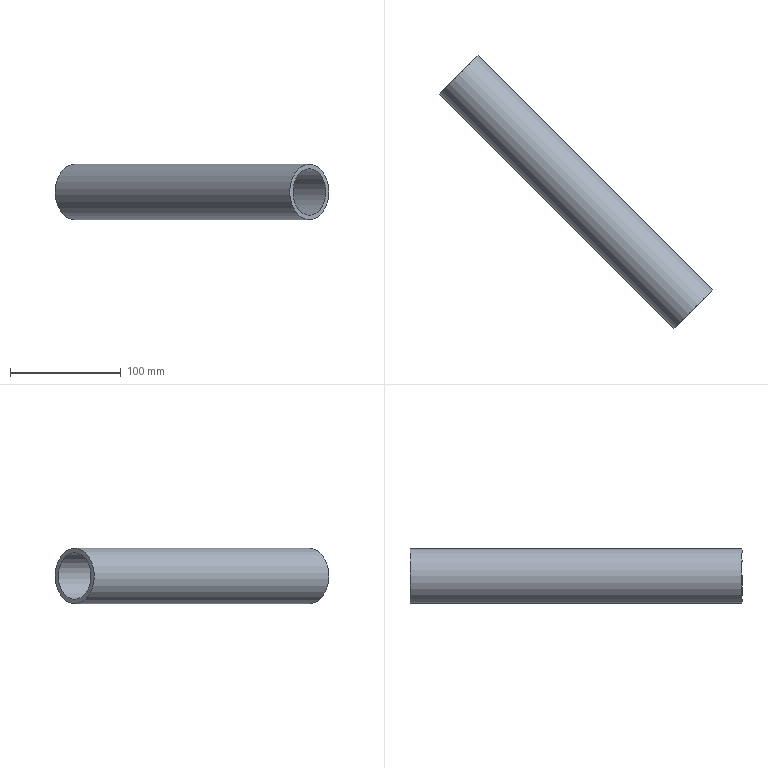Component | NX | SLID_FRAME_CONN_COL2 | 1 solid | 4 faces | box 247.49 x 247.49 x 50 mm | volume 173416 mm3 | cylinder 2 | plane 2 | commonest cylinder face diameters 50 x1 42 x1
STEP:
#1=CARTESIAN_POINT('',(0.,0.,0.));
#2=DIRECTION('',(0.,0.,1.));
#3=DIRECTION('',(1.,0.,0.));
#4=AXIS2_PLACEMENT_3D('',#1,#2,#3);
#5=CARTESIAN_POINT('',(-900.214,1525.378,235.));
#6=VERTEX_POINT('',#5);
#7=CARTESIAN_POINT('',(-900.214,1525.378,260.));
#8=DIRECTION('',(0.7071,-0.7071,0.));
#9=DIRECTION('',(0.,0.,-1.));
#10=AXIS2_PLACEMENT_3D('',#7,#8,#9);
#11=CIRCLE('',#10,25.);
#12=CARTESIAN_POINT('',(-900.214,1525.378,260.));
#13=DIRECTION('',(0.7071,-0.7071,0.));
#14=DIRECTION('',(0.,0.,1.));
#15=AXIS2_PLACEMENT_3D('',#12,#13,#14);
#16=CYLINDRICAL_SURFACE('',#15,25.);
#17=CARTESIAN_POINT('',(3.142,0.));
#18=DIRECTION('',(1.,0.));
#19=VECTOR('',#18,1.);
#20=LINE('',#17,#19);
#21=(GEOMETRIC_REPRESENTATION_CONTEXT(2)PARAMETRIC_REPRESENTATION_CONTEXT()REPRESENTATION_CONTEXT('',''));
#22=DEFINITIONAL_REPRESENTATION('',(#20),#21);
#23=PCURVE('',#16,#22);
#24=CARTESIAN_POINT('',(-900.214,1525.378,260.));
#25=DIRECTION('',(0.7071,-0.7071,0.));
#26=DIRECTION('',(0.,0.,1.));
#27=AXIS2_PLACEMENT_3D('',#24,#25,#26);
#28=PLANE('',#27);
#29=CARTESIAN_POINT('',(0.,0.));
#30=DIRECTION('',(-1.,0.));
#31=AXIS2_PLACEMENT_2D('',#29,#30);
#32=CIRCLE('',#31,25.);
#33=(GEOMETRIC_REPRESENTATION_CONTEXT(2)PARAMETRIC_REPRESENTATION_CONTEXT()REPRESENTATION_CONTEXT('',''));
#34=DEFINITIONAL_REPRESENTATION('',(#32),#33);
#35=PCURVE('',#28,#34);
#36=SURFACE_CURVE('',#11,(#23,#35),.PCURVE_S1.);
#37=EDGE_CURVE('',#6,#6,#36,.T.);
#38=ORIENTED_EDGE('',*,*,#37,.T.);
#39=CARTESIAN_POINT('',(-688.082,1313.246,235.));
#40=VERTEX_POINT('',#39);
#41=CARTESIAN_POINT('',(-900.214,1525.378,235.));
#42=CARTESIAN_POINT('',(-688.082,1313.246,235.));
#43=B_SPLINE_CURVE_WITH_KNOTS('',1,(#41,#42),.UNSPECIFIED.,.F.,.F.,(2,2),(0.,300.),.PIECEWISE_BEZIER_KNOTS.);
#44=CARTESIAN_POINT('',(9.425,0.));
#45=DIRECTION('',(0.,1.));
#46=VECTOR('',#45,1.);
#47=LINE('',#44,#46);
#48=(GEOMETRIC_REPRESENTATION_CONTEXT(2)PARAMETRIC_REPRESENTATION_CONTEXT()REPRESENTATION_CONTEXT('',''));
#49=DEFINITIONAL_REPRESENTATION('',(#47),#48);
#50=PCURVE('',#16,#49);
#51=CARTESIAN_POINT('',(3.142,0.));
#52=DIRECTION('',(0.,1.));
#53=VECTOR('',#52,1.);
#54=LINE('',#51,#53);
#55=(GEOMETRIC_REPRESENTATION_CONTEXT(2)PARAMETRIC_REPRESENTATION_CONTEXT()REPRESENTATION_CONTEXT('',''));
#56=DEFINITIONAL_REPRESENTATION('',(#54),#55);
#57=PCURVE('',#16,#56);
#58=SEAM_CURVE('',#43,(#50,#57),.PCURVE_S1.);
#59=EDGE_CURVE('',#6,#40,#58,.T.);
#60=ORIENTED_EDGE('',*,*,#59,.T.);
#61=CARTESIAN_POINT('',(-688.082,1313.246,260.));
#62=DIRECTION('',(0.7071,-0.7071,0.));
#63=DIRECTION('',(0.,0.,-1.));
#64=AXIS2_PLACEMENT_3D('',#61,#62,#63);
#65=CIRCLE('',#64,25.);
#66=CARTESIAN_POINT('',(3.142,300.));
#67=DIRECTION('',(1.,0.));
#68=VECTOR('',#67,1.);
#69=LINE('',#66,#68);
#70=(GEOMETRIC_REPRESENTATION_CONTEXT(2)PARAMETRIC_REPRESENTATION_CONTEXT()REPRESENTATION_CONTEXT('',''));
#71=DEFINITIONAL_REPRESENTATION('',(#69),#70);
#72=PCURVE('',#16,#71);
#73=CARTESIAN_POINT('',(-688.082,1313.246,260.));
#74=DIRECTION('',(0.7071,-0.7071,0.));
#75=DIRECTION('',(0.,0.,1.));
#76=AXIS2_PLACEMENT_3D('',#73,#74,#75);
#77=PLANE('',#76);
#78=CARTESIAN_POINT('',(0.,0.));
#79=DIRECTION('',(-1.,0.));
#80=AXIS2_PLACEMENT_2D('',#78,#79);
#81=CIRCLE('',#80,25.);
#82=(GEOMETRIC_REPRESENTATION_CONTEXT(2)PARAMETRIC_REPRESENTATION_CONTEXT()REPRESENTATION_CONTEXT('',''));
#83=DEFINITIONAL_REPRESENTATION('',(#81),#82);
#84=PCURVE('',#77,#83);
#85=SURFACE_CURVE('',#65,(#72,#84),.PCURVE_S1.);
#86=EDGE_CURVE('',#40,#40,#85,.T.);
#87=ORIENTED_EDGE('',*,*,#86,.F.);
#88=ORIENTED_EDGE('',*,*,#59,.F.);
#89=EDGE_LOOP('',(#38,#60,#87,#88));
#90=FACE_BOUND('',#89,.T.);
#91=ADVANCED_FACE('',(#90),#16,.T.);
#92=CARTESIAN_POINT('',(-900.214,1525.378,239.));
#93=VERTEX_POINT('',#92);
#94=CARTESIAN_POINT('',(-900.214,1525.378,260.));
#95=DIRECTION('',(0.7071,-0.7071,0.));
#96=DIRECTION('',(0.,0.,-1.));
#97=AXIS2_PLACEMENT_3D('',#94,#95,#96);
#98=CIRCLE('',#97,21.);
#99=CARTESIAN_POINT('',(-900.214,1525.378,260.));
#100=DIRECTION('',(0.7071,-0.7071,0.));
#101=DIRECTION('',(0.,0.,1.));
#102=AXIS2_PLACEMENT_3D('',#99,#100,#101);
#103=CYLINDRICAL_SURFACE('',#102,21.);
#104=CARTESIAN_POINT('',(3.142,0.));
#105=DIRECTION('',(1.,0.));
#106=VECTOR('',#105,1.);
#107=LINE('',#104,#106);
#108=(GEOMETRIC_REPRESENTATION_CONTEXT(2)PARAMETRIC_REPRESENTATION_CONTEXT()REPRESENTATION_CONTEXT('',''));
#109=DEFINITIONAL_REPRESENTATION('',(#107),#108);
#110=PCURVE('',#103,#109);
#111=CARTESIAN_POINT('',(0.,0.));
#112=DIRECTION('',(-1.,0.));
#113=AXIS2_PLACEMENT_2D('',#111,#112);
#114=CIRCLE('',#113,21.);
#115=(GEOMETRIC_REPRESENTATION_CONTEXT(2)PARAMETRIC_REPRESENTATION_CONTEXT()REPRESENTATION_CONTEXT('',''));
#116=DEFINITIONAL_REPRESENTATION('',(#114),#115);
#117=PCURVE('',#28,#116);
#118=SURFACE_CURVE('',#98,(#110,#117),.PCURVE_S1.);
#119=EDGE_CURVE('',#93,#93,#118,.T.);
#120=ORIENTED_EDGE('',*,*,#119,.T.);
#121=CARTESIAN_POINT('',(-688.082,1313.246,239.));
#122=VERTEX_POINT('',#121);
#123=CARTESIAN_POINT('',(-900.214,1525.378,239.));
#124=CARTESIAN_POINT('',(-688.082,1313.246,239.));
#125=B_SPLINE_CURVE_WITH_KNOTS('',1,(#123,#124),.UNSPECIFIED.,.F.,.F.,(2,2),(0.,300.),.PIECEWISE_BEZIER_KNOTS.);
#126=CARTESIAN_POINT('',(9.425,0.));
#127=DIRECTION('',(0.,1.));
#128=VECTOR('',#127,1.);
#129=LINE('',#126,#128);
#130=(GEOMETRIC_REPRESENTATION_CONTEXT(2)PARAMETRIC_REPRESENTATION_CONTEXT()REPRESENTATION_CONTEXT('',''));
#131=DEFINITIONAL_REPRESENTATION('',(#129),#130);
#132=PCURVE('',#103,#131);
#133=CARTESIAN_POINT('',(3.142,0.));
#134=DIRECTION('',(0.,1.));
#135=VECTOR('',#134,1.);
#136=LINE('',#133,#135);
#137=(GEOMETRIC_REPRESENTATION_CONTEXT(2)PARAMETRIC_REPRESENTATION_CONTEXT()REPRESENTATION_CONTEXT('',''));
#138=DEFINITIONAL_REPRESENTATION('',(#136),#137);
#139=PCURVE('',#103,#138);
#140=SEAM_CURVE('',#125,(#132,#139),.PCURVE_S1.);
#141=EDGE_CURVE('',#93,#122,#140,.T.);
#142=ORIENTED_EDGE('',*,*,#141,.T.);
#143=CARTESIAN_POINT('',(-688.082,1313.246,260.));
#144=DIRECTION('',(0.7071,-0.7071,0.));
#145=DIRECTION('',(0.,0.,-1.));
#146=AXIS2_PLACEMENT_3D('',#143,#144,#145);
#147=CIRCLE('',#146,21.);
#148=CARTESIAN_POINT('',(3.142,300.));
#149=DIRECTION('',(1.,0.));
#150=VECTOR('',#149,1.);
#151=LINE('',#148,#150);
#152=(GEOMETRIC_REPRESENTATION_CONTEXT(2)PARAMETRIC_REPRESENTATION_CONTEXT()REPRESENTATION_CONTEXT('',''));
#153=DEFINITIONAL_REPRESENTATION('',(#151),#152);
#154=PCURVE('',#103,#153);
#155=CARTESIAN_POINT('',(0.,0.));
#156=DIRECTION('',(-1.,0.));
#157=AXIS2_PLACEMENT_2D('',#155,#156);
#158=CIRCLE('',#157,21.);
#159=(GEOMETRIC_REPRESENTATION_CONTEXT(2)PARAMETRIC_REPRESENTATION_CONTEXT()REPRESENTATION_CONTEXT('',''));
#160=DEFINITIONAL_REPRESENTATION('',(#158),#159);
#161=PCURVE('',#77,#160);
#162=SURFACE_CURVE('',#147,(#154,#161),.PCURVE_S1.);
#163=EDGE_CURVE('',#122,#122,#162,.T.);
#164=ORIENTED_EDGE('',*,*,#163,.F.);
#165=ORIENTED_EDGE('',*,*,#141,.F.);
#166=EDGE_LOOP('',(#120,#142,#164,#165));
#167=FACE_BOUND('',#166,.F.);
#168=ADVANCED_FACE('',(#167),#103,.F.);
#169=ORIENTED_EDGE('',*,*,#37,.F.);
#170=EDGE_LOOP('',(#169));
#171=FACE_BOUND('',#170,.T.);
#172=ORIENTED_EDGE('',*,*,#119,.T.);
#173=EDGE_LOOP('',(#172));
#174=FACE_BOUND('',#173,.T.);
#175=ADVANCED_FACE('',(#171,#174),#28,.F.);
#176=ORIENTED_EDGE('',*,*,#86,.T.);
#177=EDGE_LOOP('',(#176));
#178=FACE_BOUND('',#177,.T.);
#179=ORIENTED_EDGE('',*,*,#163,.F.);
#180=EDGE_LOOP('',(#179));
#181=FACE_BOUND('',#180,.T.);
#182=ADVANCED_FACE('',(#178,#181),#77,.T.);
#183=CLOSED_SHELL('',(#91,#168,#175,#182));
#184=MANIFOLD_SOLID_BREP('',#183);
#185=(LENGTH_UNIT()NAMED_UNIT(*)SI_UNIT(.MILLI.,.METRE.));
#186=UNCERTAINTY_MEASURE_WITH_UNIT(LENGTH_MEASURE(0.00001),#185,'','');
#187=(NAMED_UNIT(*)PLANE_ANGLE_UNIT()SI_UNIT($,.RADIAN.));
#188=(NAMED_UNIT(*)SI_UNIT($,.STERADIAN.)SOLID_ANGLE_UNIT());
#189=(GEOMETRIC_REPRESENTATION_CONTEXT(3)GLOBAL_UNCERTAINTY_ASSIGNED_CONTEXT((#186))GLOBAL_UNIT_ASSIGNED_CONTEXT((#185,#187,#188))REPRESENTATION_CONTEXT('',''));
#190=ADVANCED_BREP_SHAPE_REPRESENTATION('',(#4,#184),#189);